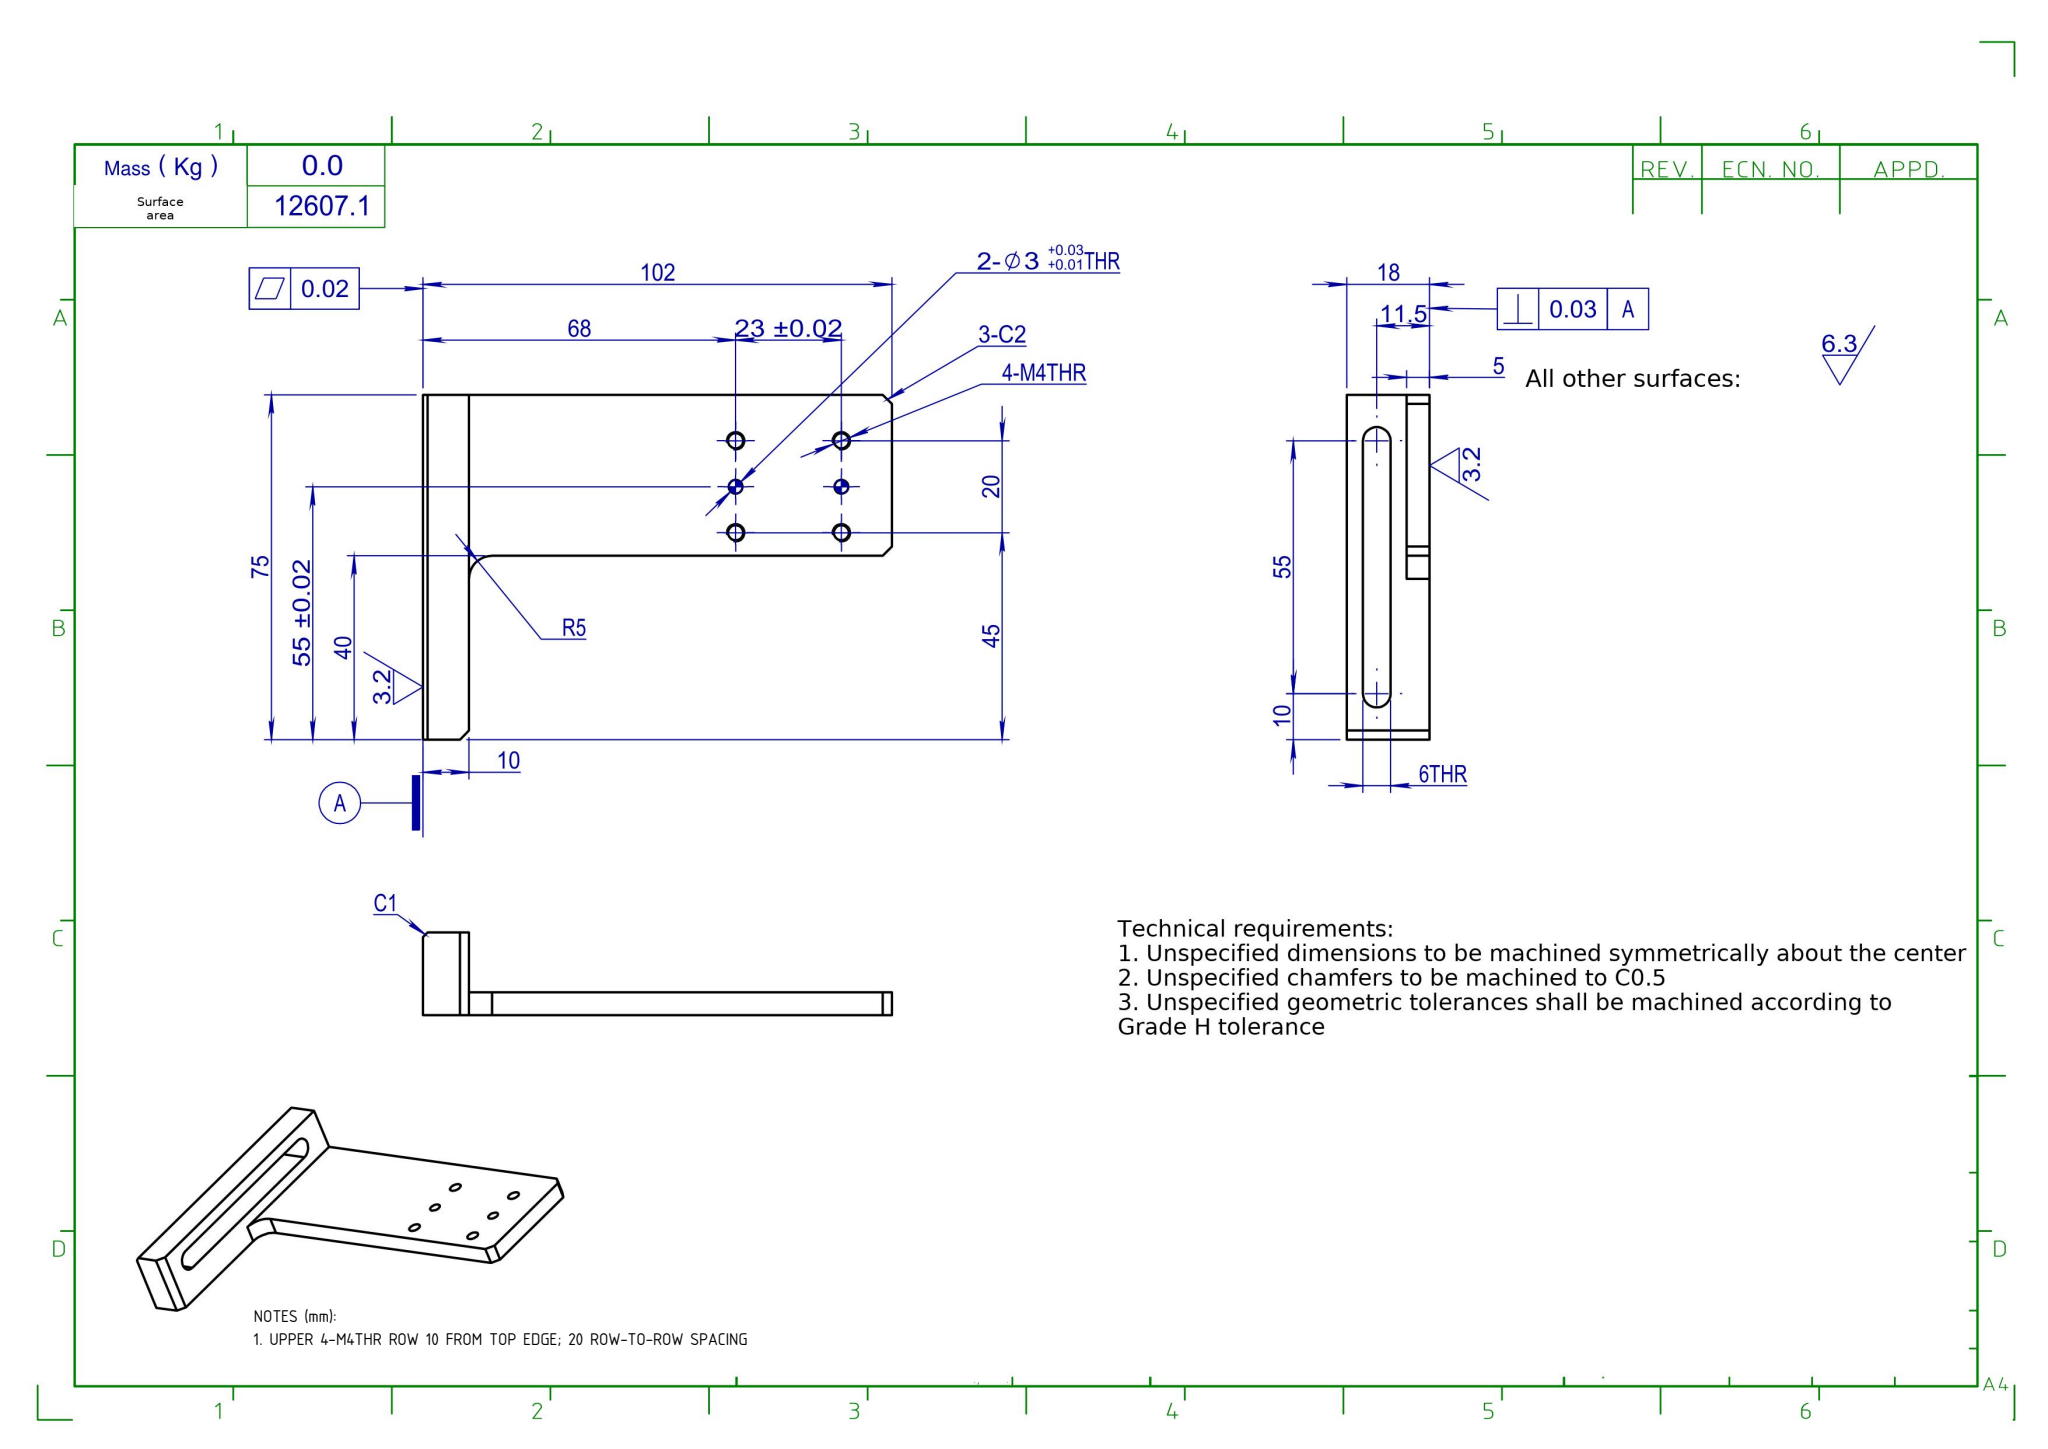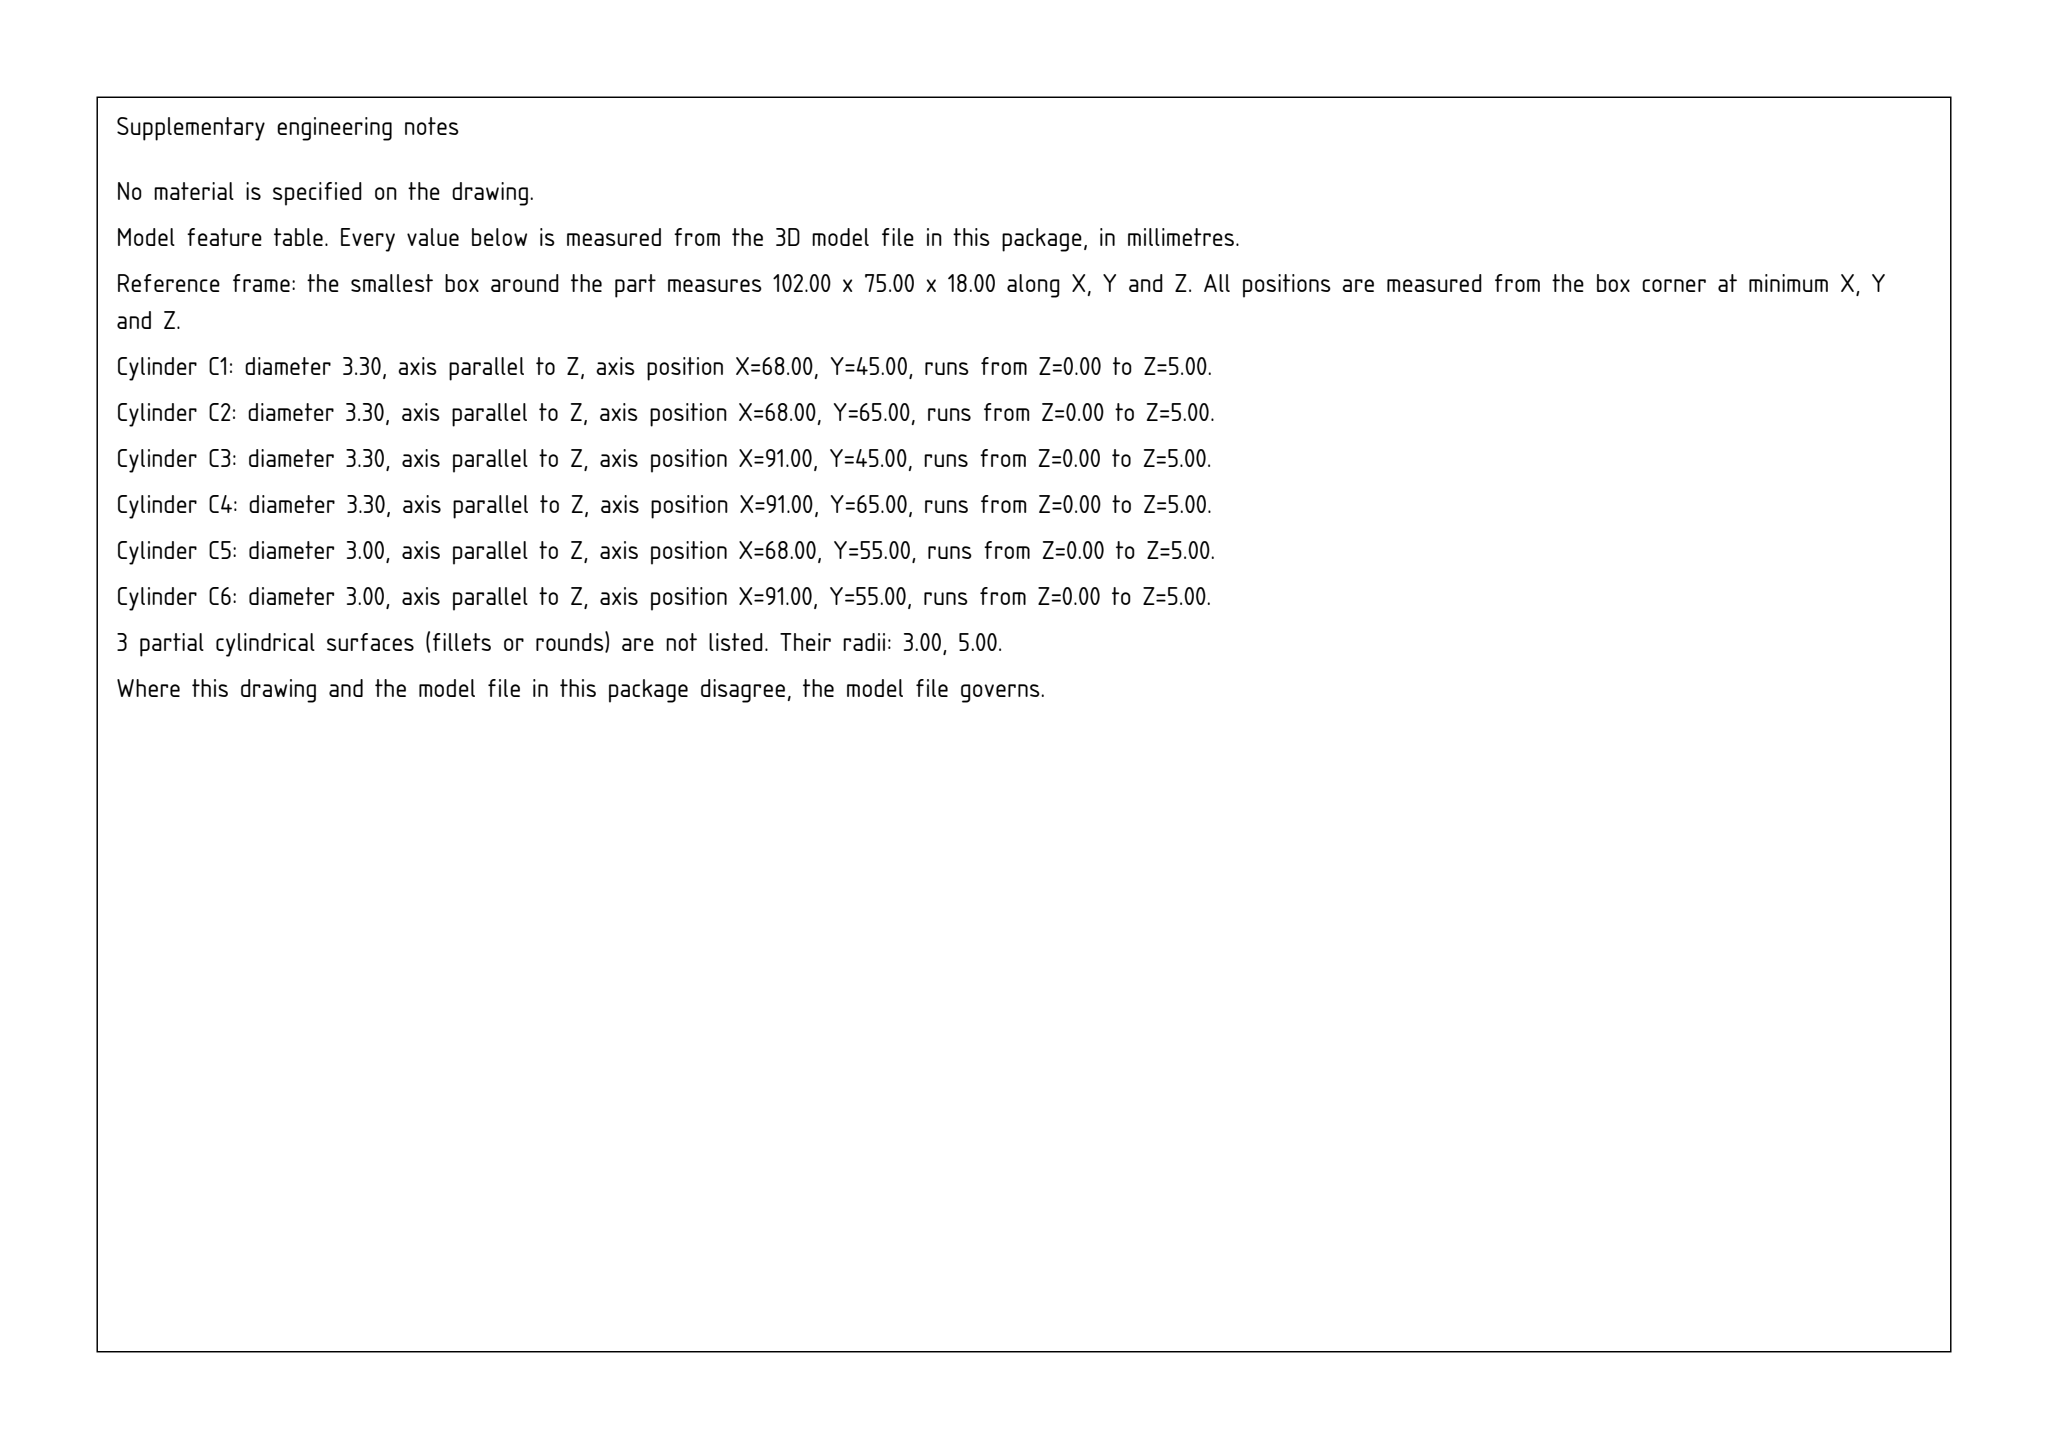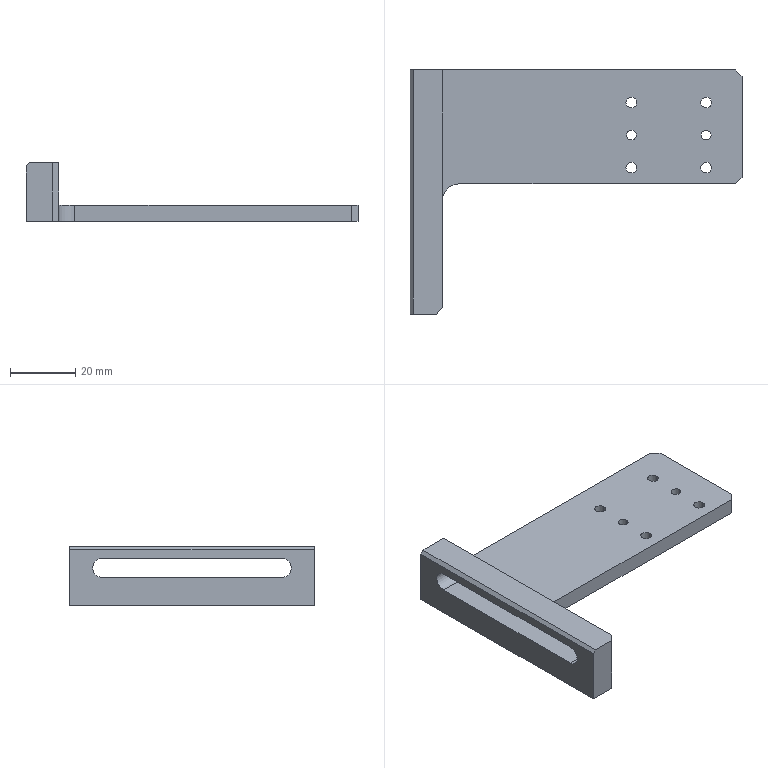Part | SolidWorks | mm | 1 solid | 30 faces | box 102 x 75 x 18 mm | volume 25709 mm3 | cylinder 15 | plane 15 | commonest cylinder face diameters 3.3 x8 3 x4 6 x2 10 x1
Drawing notes:
UPPER 4-M4THR ROW 10 FROM TOP EDGE; 20 ROW-TO-ROW SPACING | from the solid: Ø3.3 z-holes at y=65 and y=45; bbox y=75 top edge
build123d program:
from build123d import *

# Parameters (mm, degrees)
EXTRUDE1_DEPTH        = 18
FILLET1_R             = 5
CUT_EXTRUDE2_DEPTH    = 149.138
M4_TAPPED_HOLE1_D     = 3.3
M4_TAPPED_HOLE1_DEPTH = 11.5
M4_TAPPED_HOLE1_TIP   = 0.9914
CHAMFER1_SIZE         = 2
SKETCH9_R             = 1.5
CUT_EXTRUDE4_DEPTH    = 112.032
SKETCH10_W            = 92
SKETCH10_H            = 50
CUT_EXTRUDE5_DEPTH    = 13
CHAMFER2_SIZE         = 1


with BuildPart() as part:
    # Sketch1 → Extrude1 (new body)
    with BuildSketch(Plane.XY):
        Polygon((-92, 0), (-92, -40), (-102, -40), (-102, 35), (0, 35), (0, 0), align=None)
    extrude(amount=EXTRUDE1_DEPTH)

    # Fillet1
    fillet1_edges = [part.edges().sort_by_distance(p)[0] for p in [
        (-92, 0, 9),
    ]]
    fillet(fillet1_edges, radius=FILLET1_R)

    # Sketch3 → Cut-Extrude2 (cut, through all)
    with BuildSketch(Plane(origin=(-92, 0, -91), x_dir=(0, 0, 1), z_dir=(-1, 0, 0))):
        with BuildLine():
            Line((99.5, 25), (99.5, -30))
            ThreePointArc((99.5, -30), (102.5, -33), (105.5, -30))
            Line((105.5, -30), (105.5, 25))
            ThreePointArc((105.5, 25), (102.5, 28), (99.5, 25))
        make_face()
    extrude(amount=CUT_EXTRUDE2_DEPTH, mode=Mode.SUBTRACT)

    # M4 Tapped Hole1
    with Locations(Plane(origin=(31.187, 12.711, 0), x_dir=(1, 0, 0), z_dir=(0, 0, -1))):
        with Locations((-42.187, 7.711), (-65.187, 7.711), (-65.187, -12.289), (-42.187, -12.289)):
            Hole(M4_TAPPED_HOLE1_D / 2, depth=M4_TAPPED_HOLE1_DEPTH)
            with Locations((0, 0, -(M4_TAPPED_HOLE1_DEPTH + M4_TAPPED_HOLE1_TIP / 2))):  # 118° drill point
                Cone(0, M4_TAPPED_HOLE1_D / 2, M4_TAPPED_HOLE1_TIP, mode=Mode.SUBTRACT)

    # Chamfer1
    chamfer1_edges = [part.edges().sort_by_distance(p)[0] for p in [
        (0, 0, 9),
        (-92, -40, 9),
        (0, 35, 9),
    ]]
    chamfer(chamfer1_edges, length=CHAMFER1_SIZE)

    # Sketch9 → Cut-Extrude4 (cut, through all)
    with BuildSketch(Plane.XY.offset(18)):
        with Locations((-34, 15)):
            Circle(SKETCH9_R)
        with Locations((-11, 15)):
            Circle(SKETCH9_R)
    extrude(amount=-CUT_EXTRUDE4_DEPTH, mode=Mode.SUBTRACT)

    # Sketch10 → Cut-Extrude5 (cut)
    with BuildSketch(Plane(origin=(0, 0, 18), x_dir=(-1, 0, 0), z_dir=(0, 0, -1))):
        with Locations((46, 10)):
            Rectangle(SKETCH10_W, SKETCH10_H)
    extrude(amount=CUT_EXTRUDE5_DEPTH, mode=Mode.SUBTRACT)

    # Chamfer2
    chamfer2_edges = [part.edges().sort_by_distance(p)[0] for p in [
        (-102, -2.5, 18),
    ]]
    chamfer(chamfer2_edges, length=CHAMFER2_SIZE)


solid = part.part